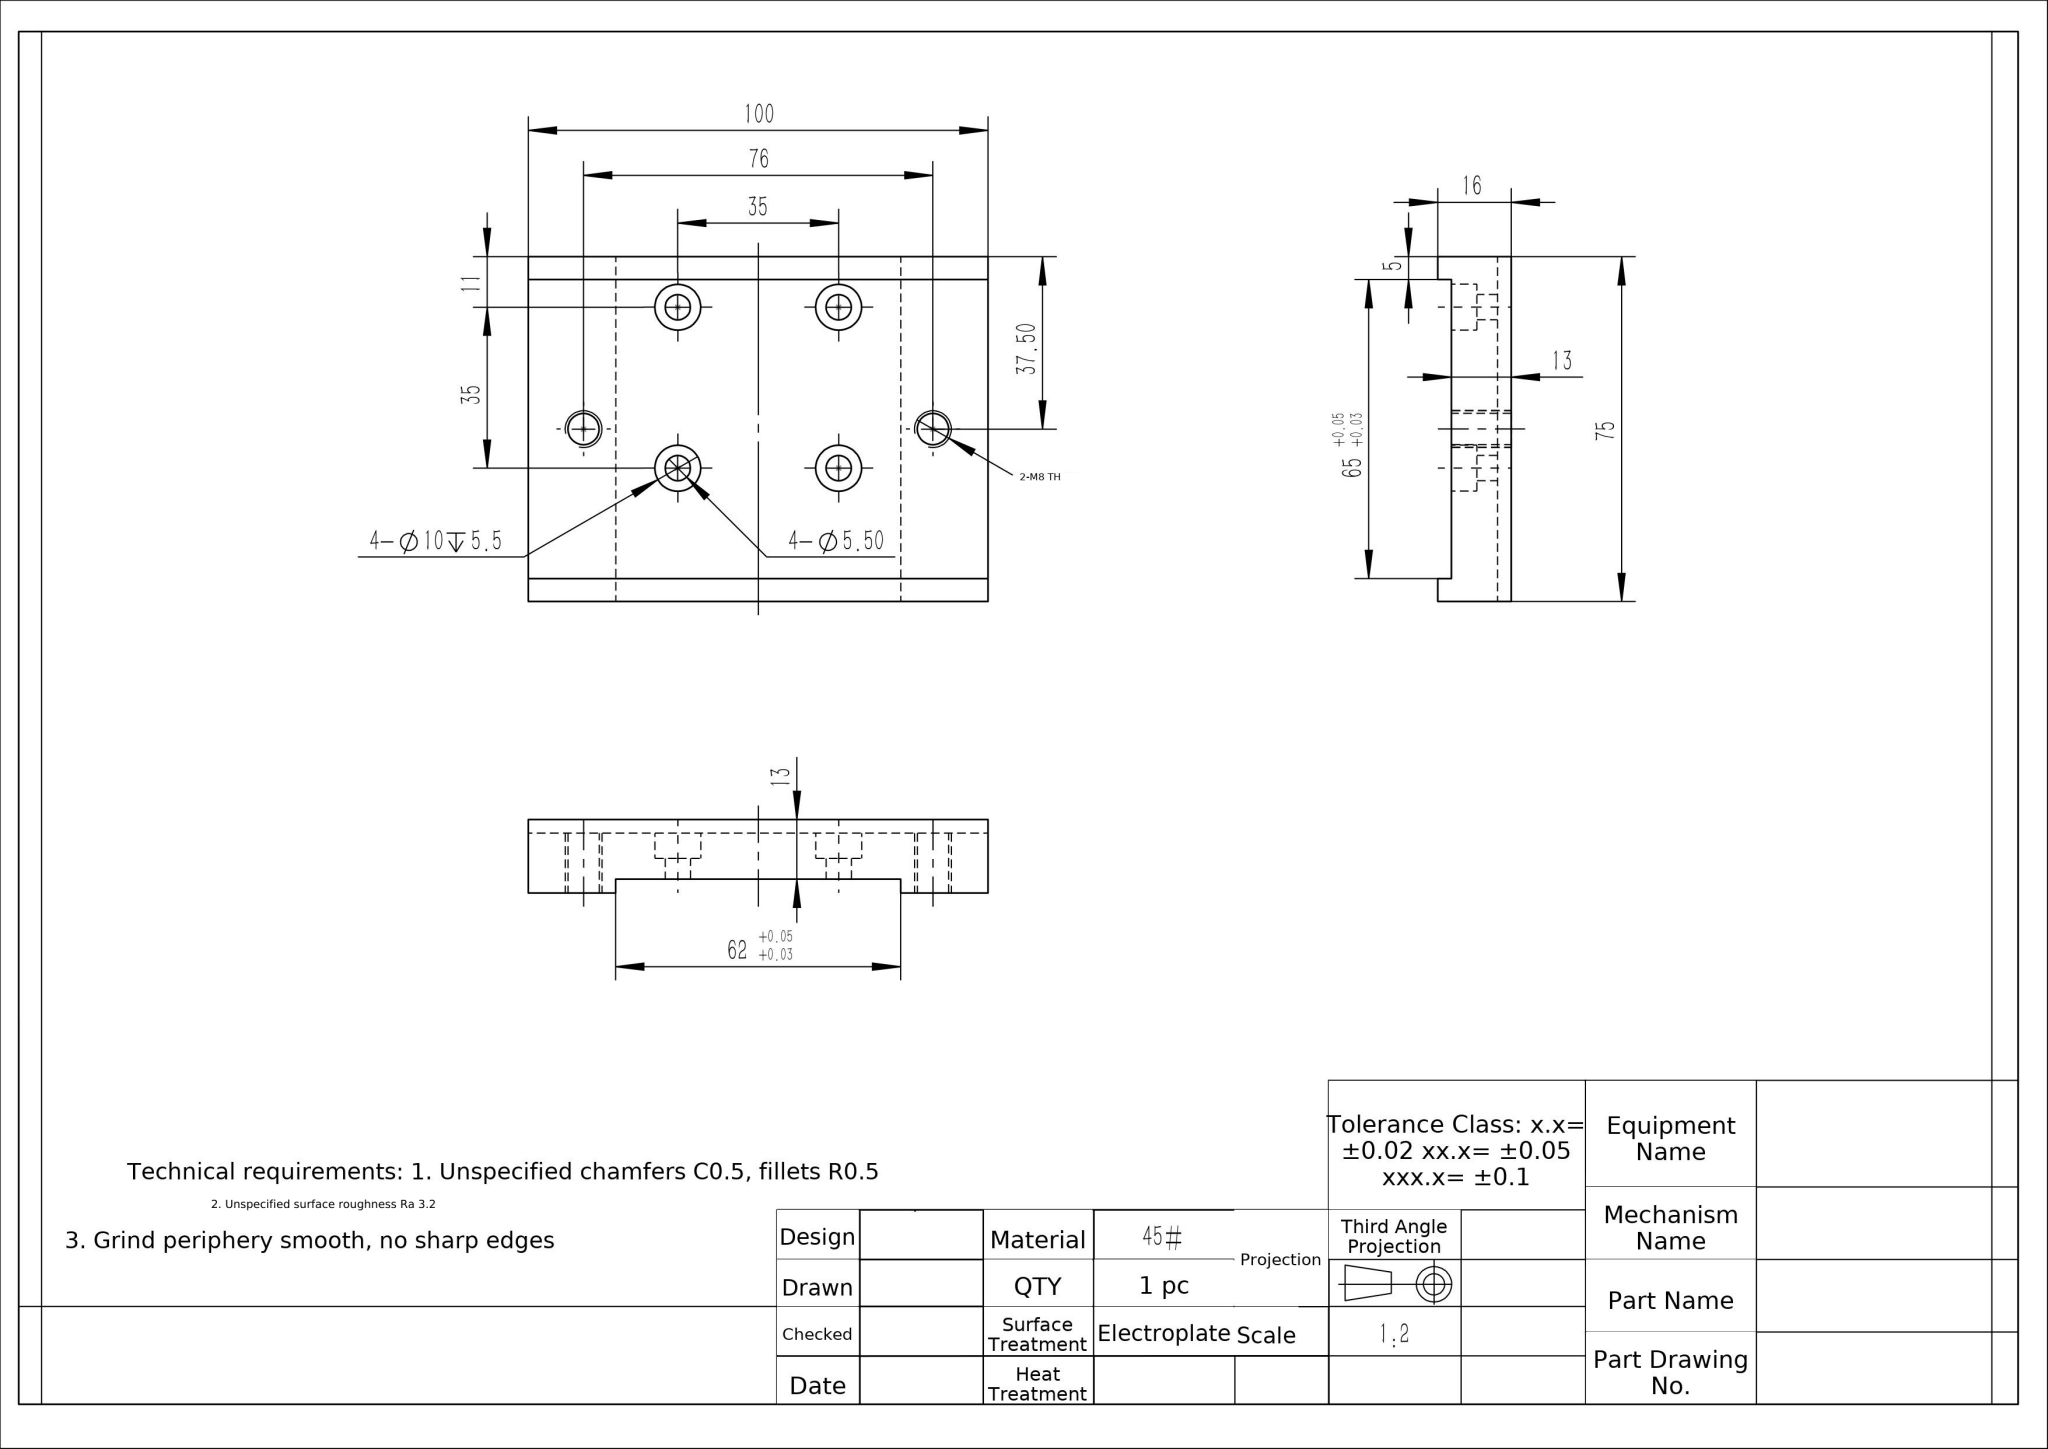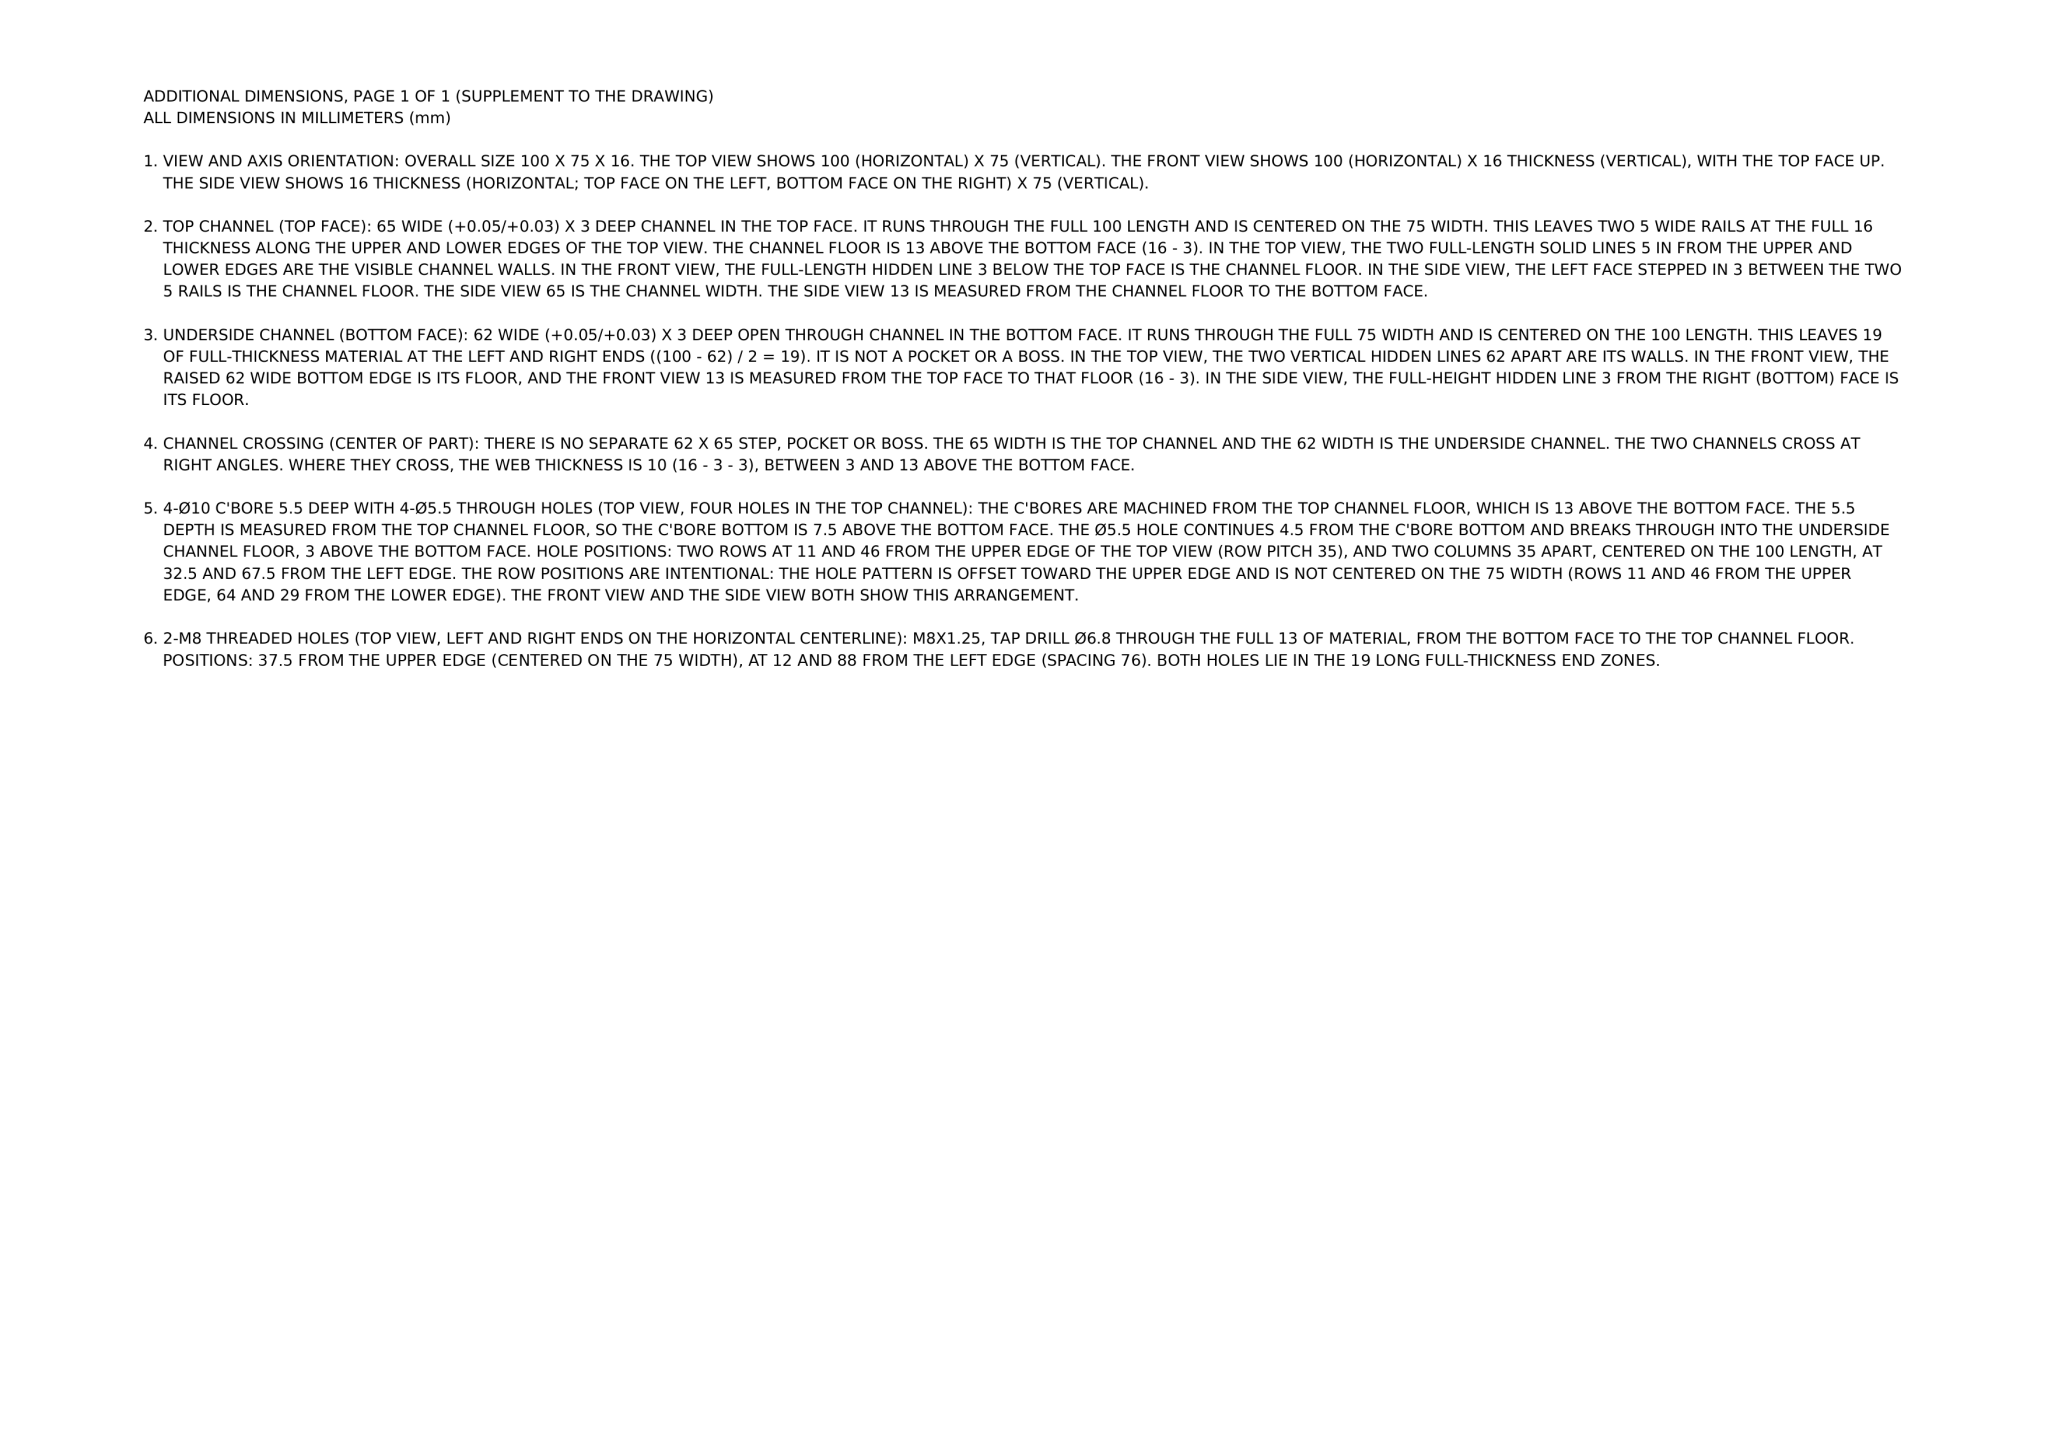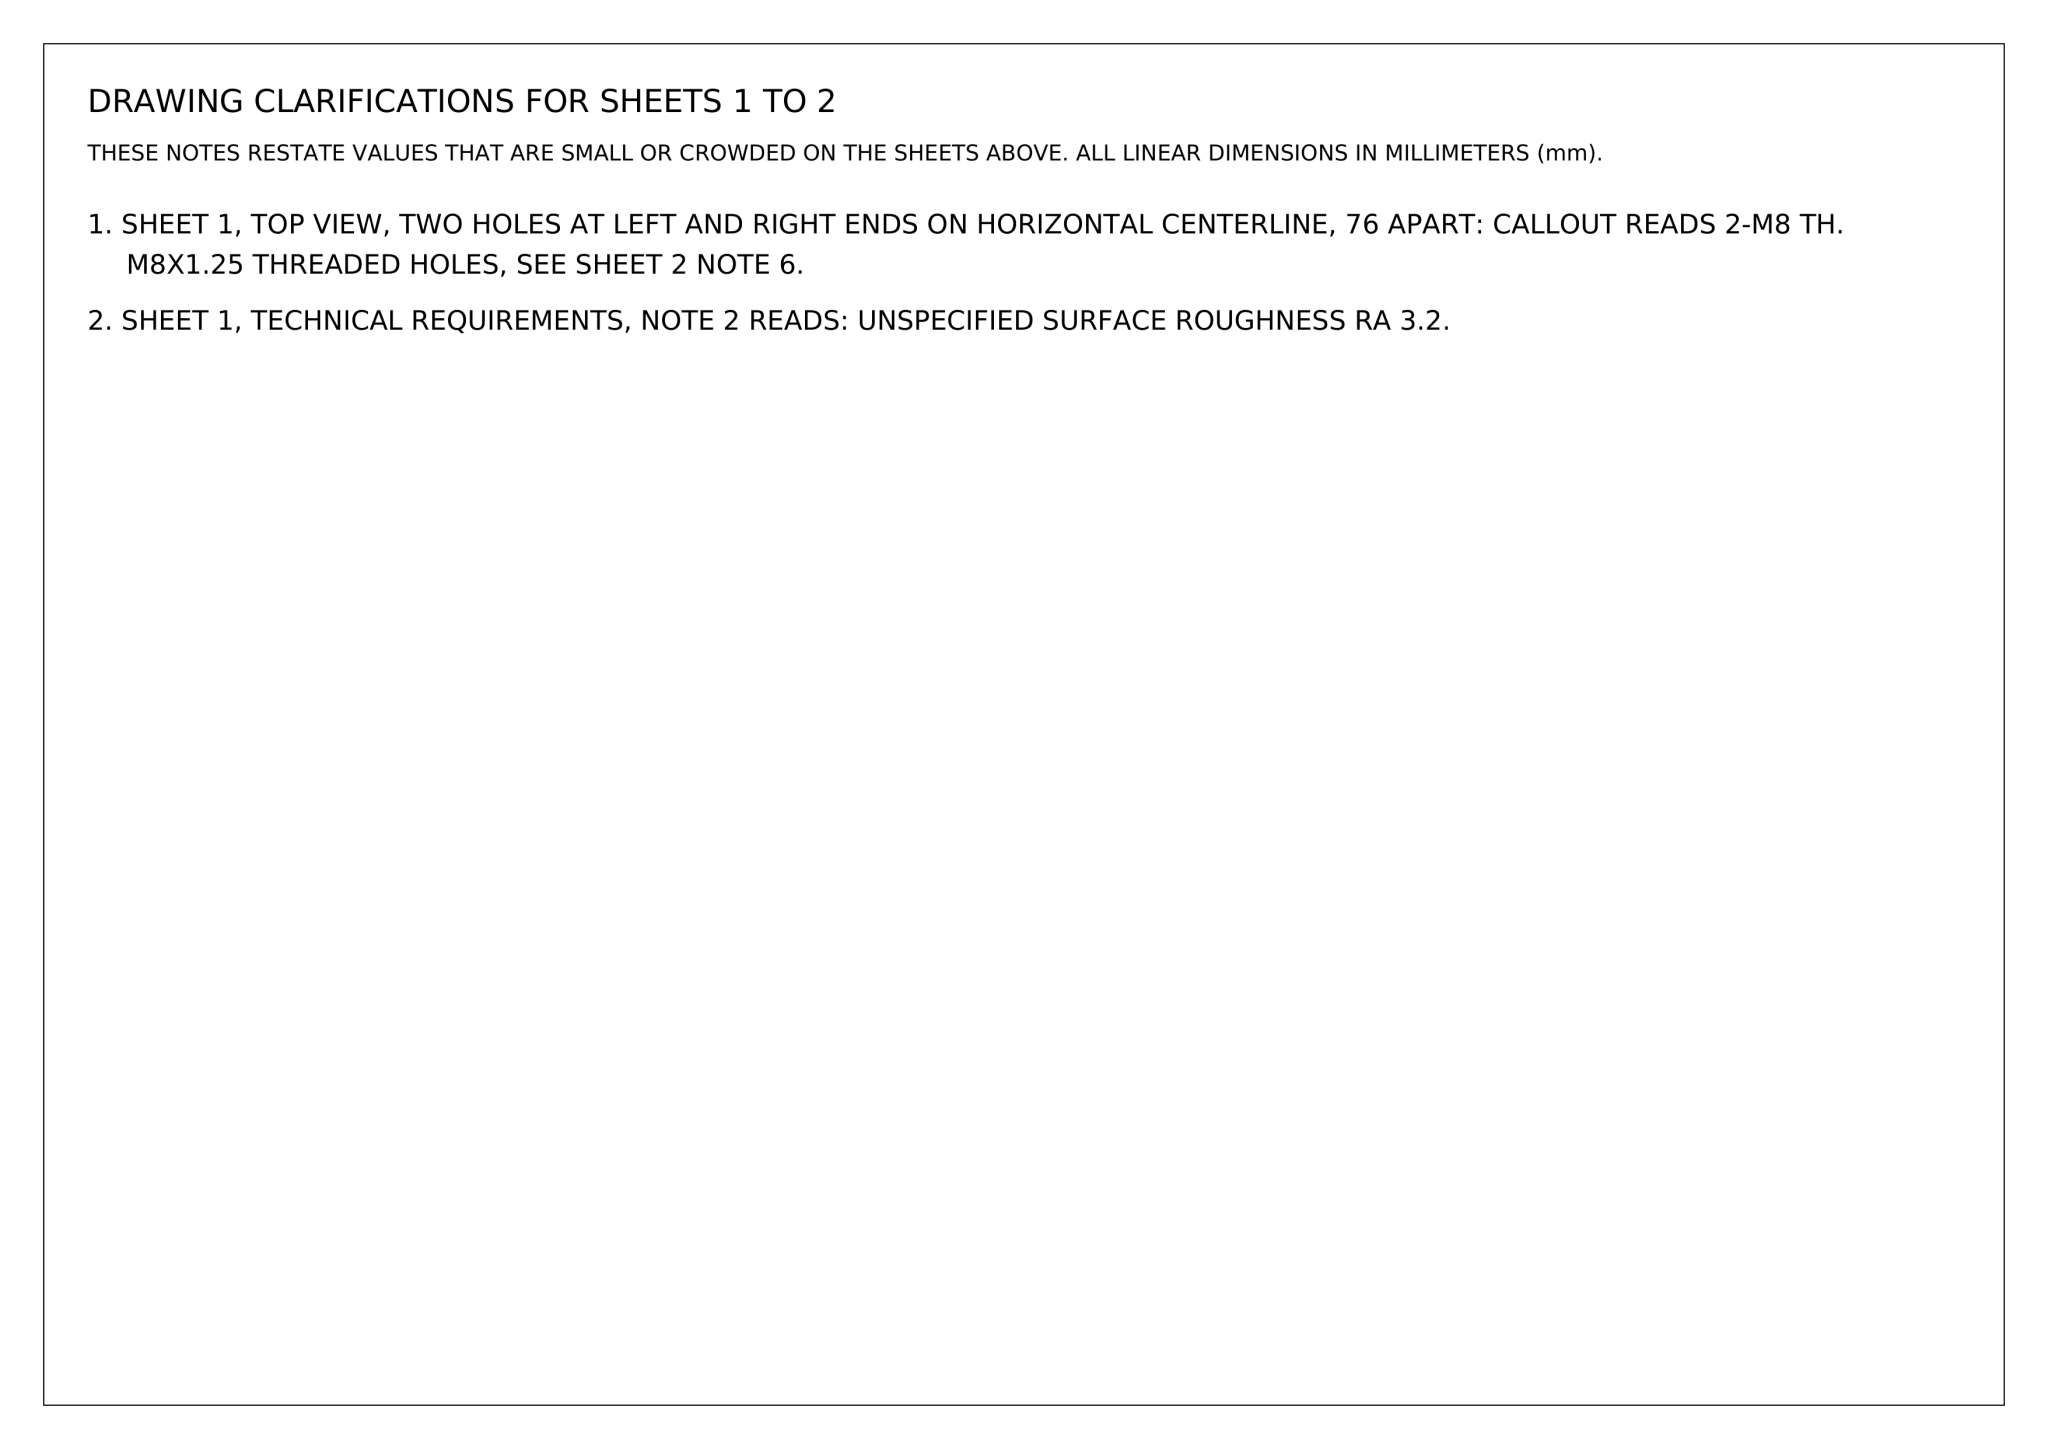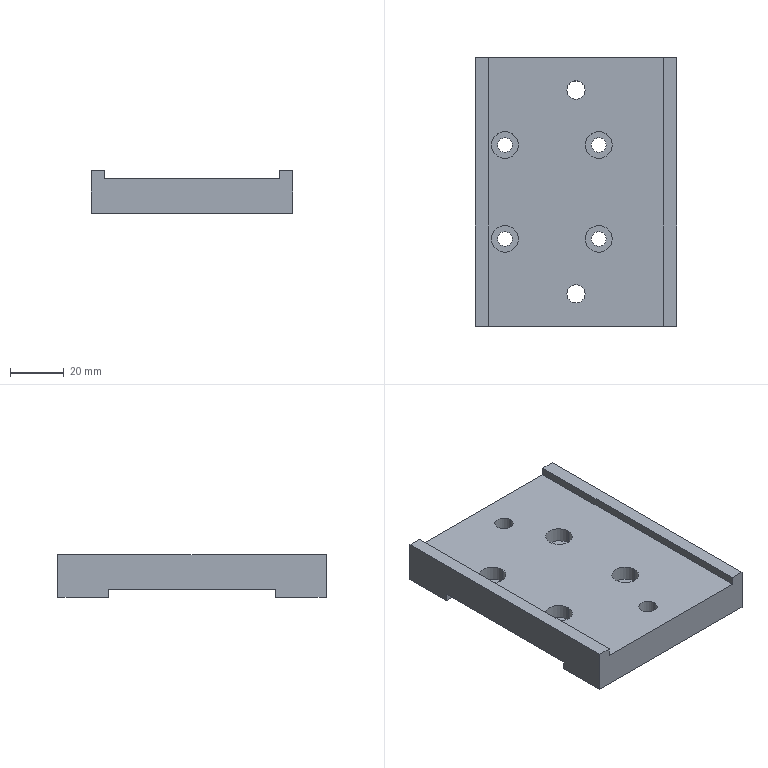Part | NX | mm | 1 solid | 38 faces | box 75 x 100 x 16 mm | volume 83450 mm3 | cylinder 20 | plane 18 | commonest cylinder face diameters 10 x8 5.5 x8 6.8 x4